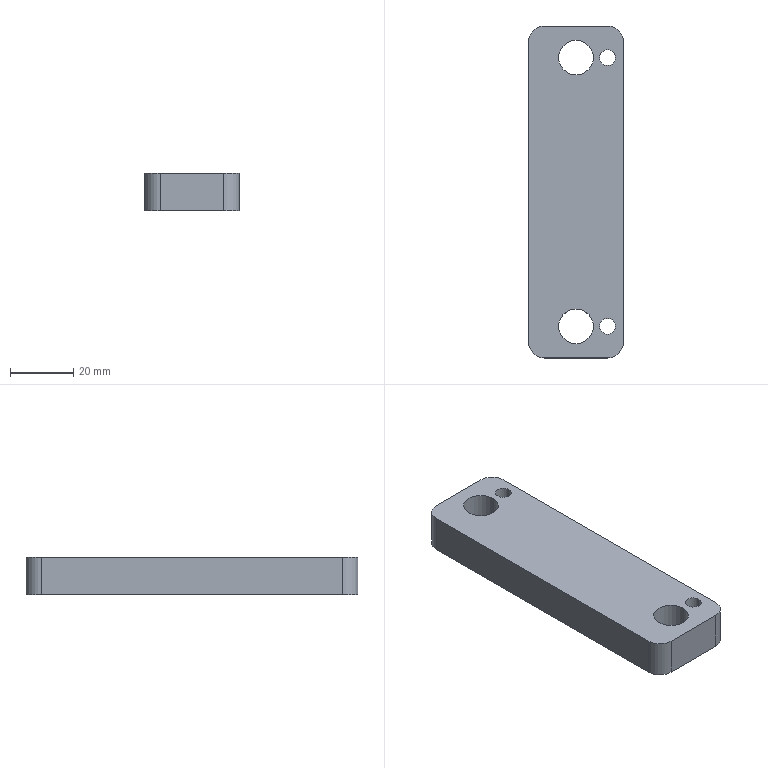CAM job | Mastercam | mm | 12 operations | part box 30 x 105 x 12
1. 2D High Speed (2D Dynamic Mill) | 8 - 8 平铣刀
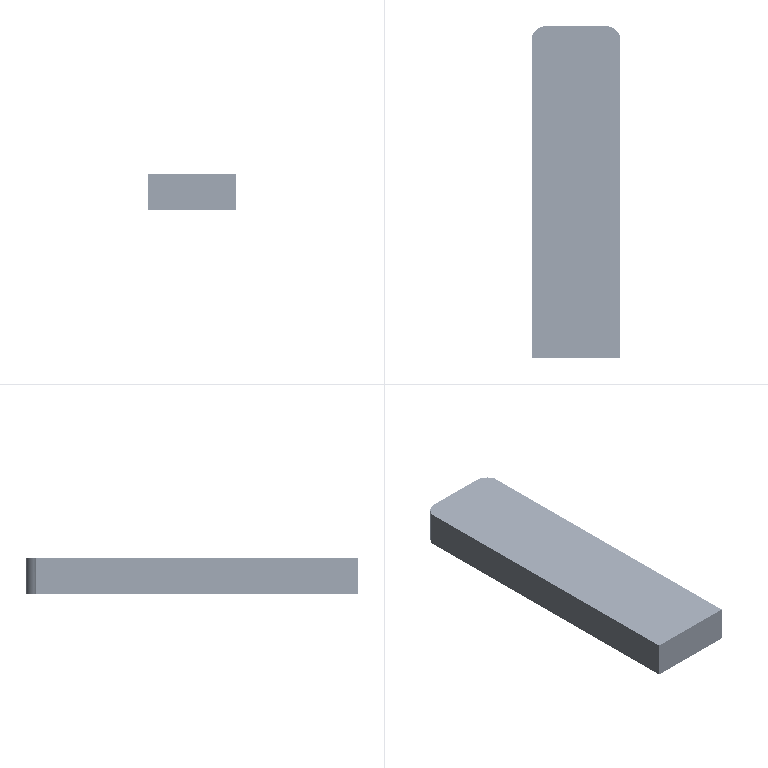2. Contour (Ramp) | 20 - 21 平铣刀
3. Drill/Counterbore | 7 - 4 倒角刀
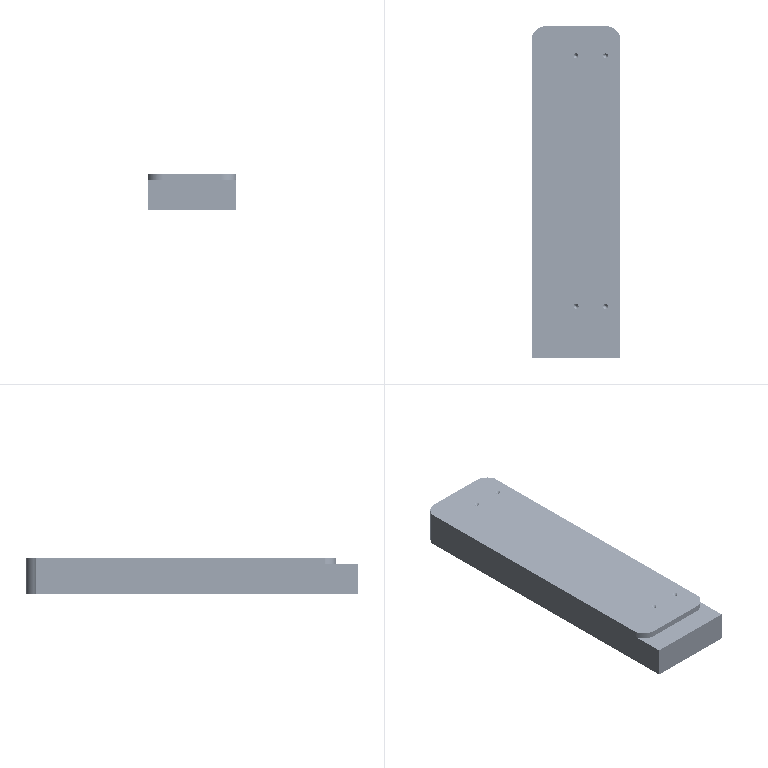4. Peck Drill | 1 - 10.5 钻头
5. Contour (Ramp) | 9 - 8 平铣刀
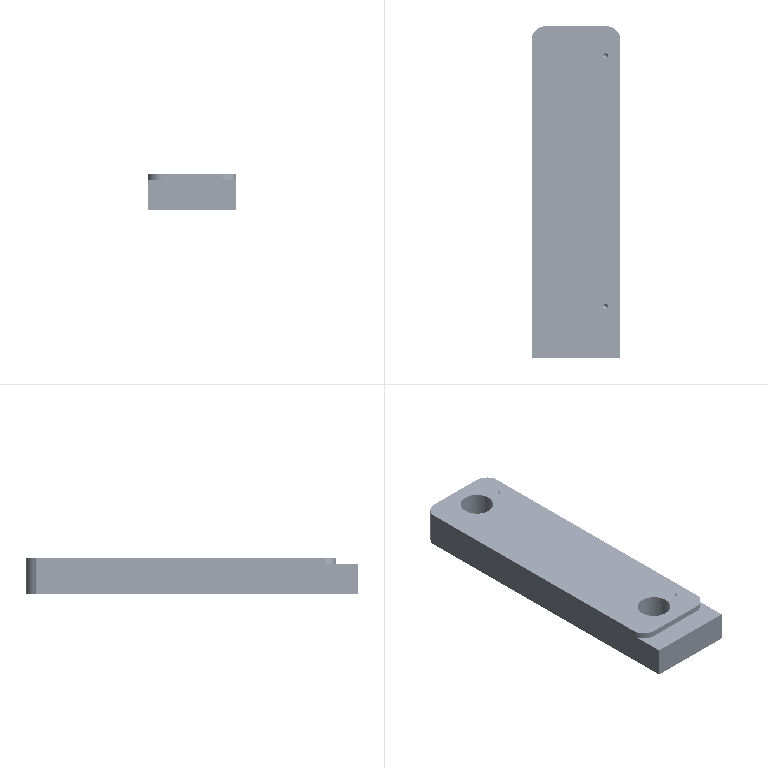6. Contour (2D) | 9 - 8 平铣刀
7. Facing | 9 - 8 平铣刀
8. Contour (2D chamfer) | 7 - 4 倒角刀
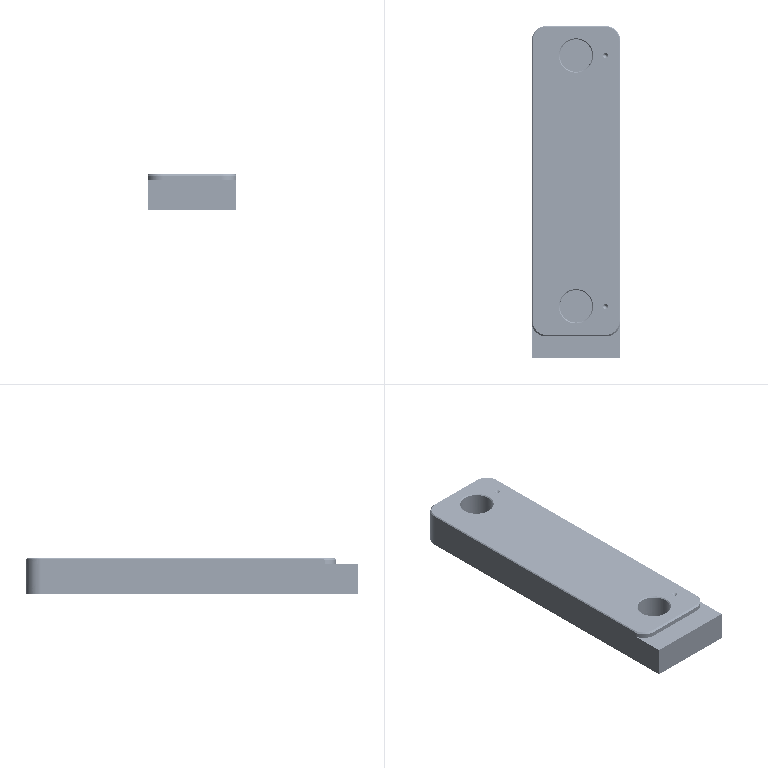9. Facing | 9 - 8 平铣刀
10. 2D High Speed (2D Dynamic Mill) | 8 - 8 平铣刀
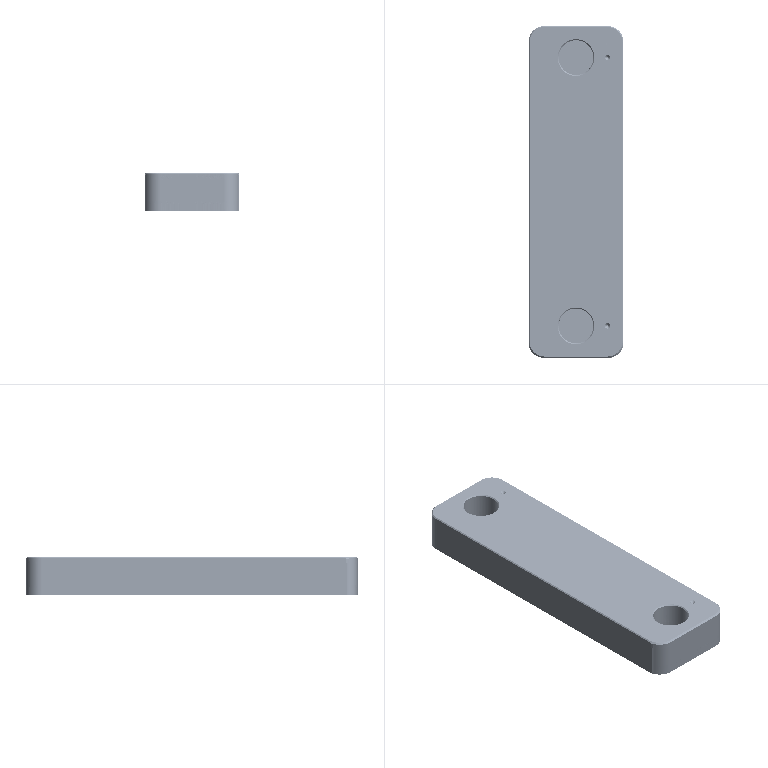11. Contour (2D) | 9 - 8 平铣刀
12. Contour (2D chamfer) | 7 - 4 倒角刀